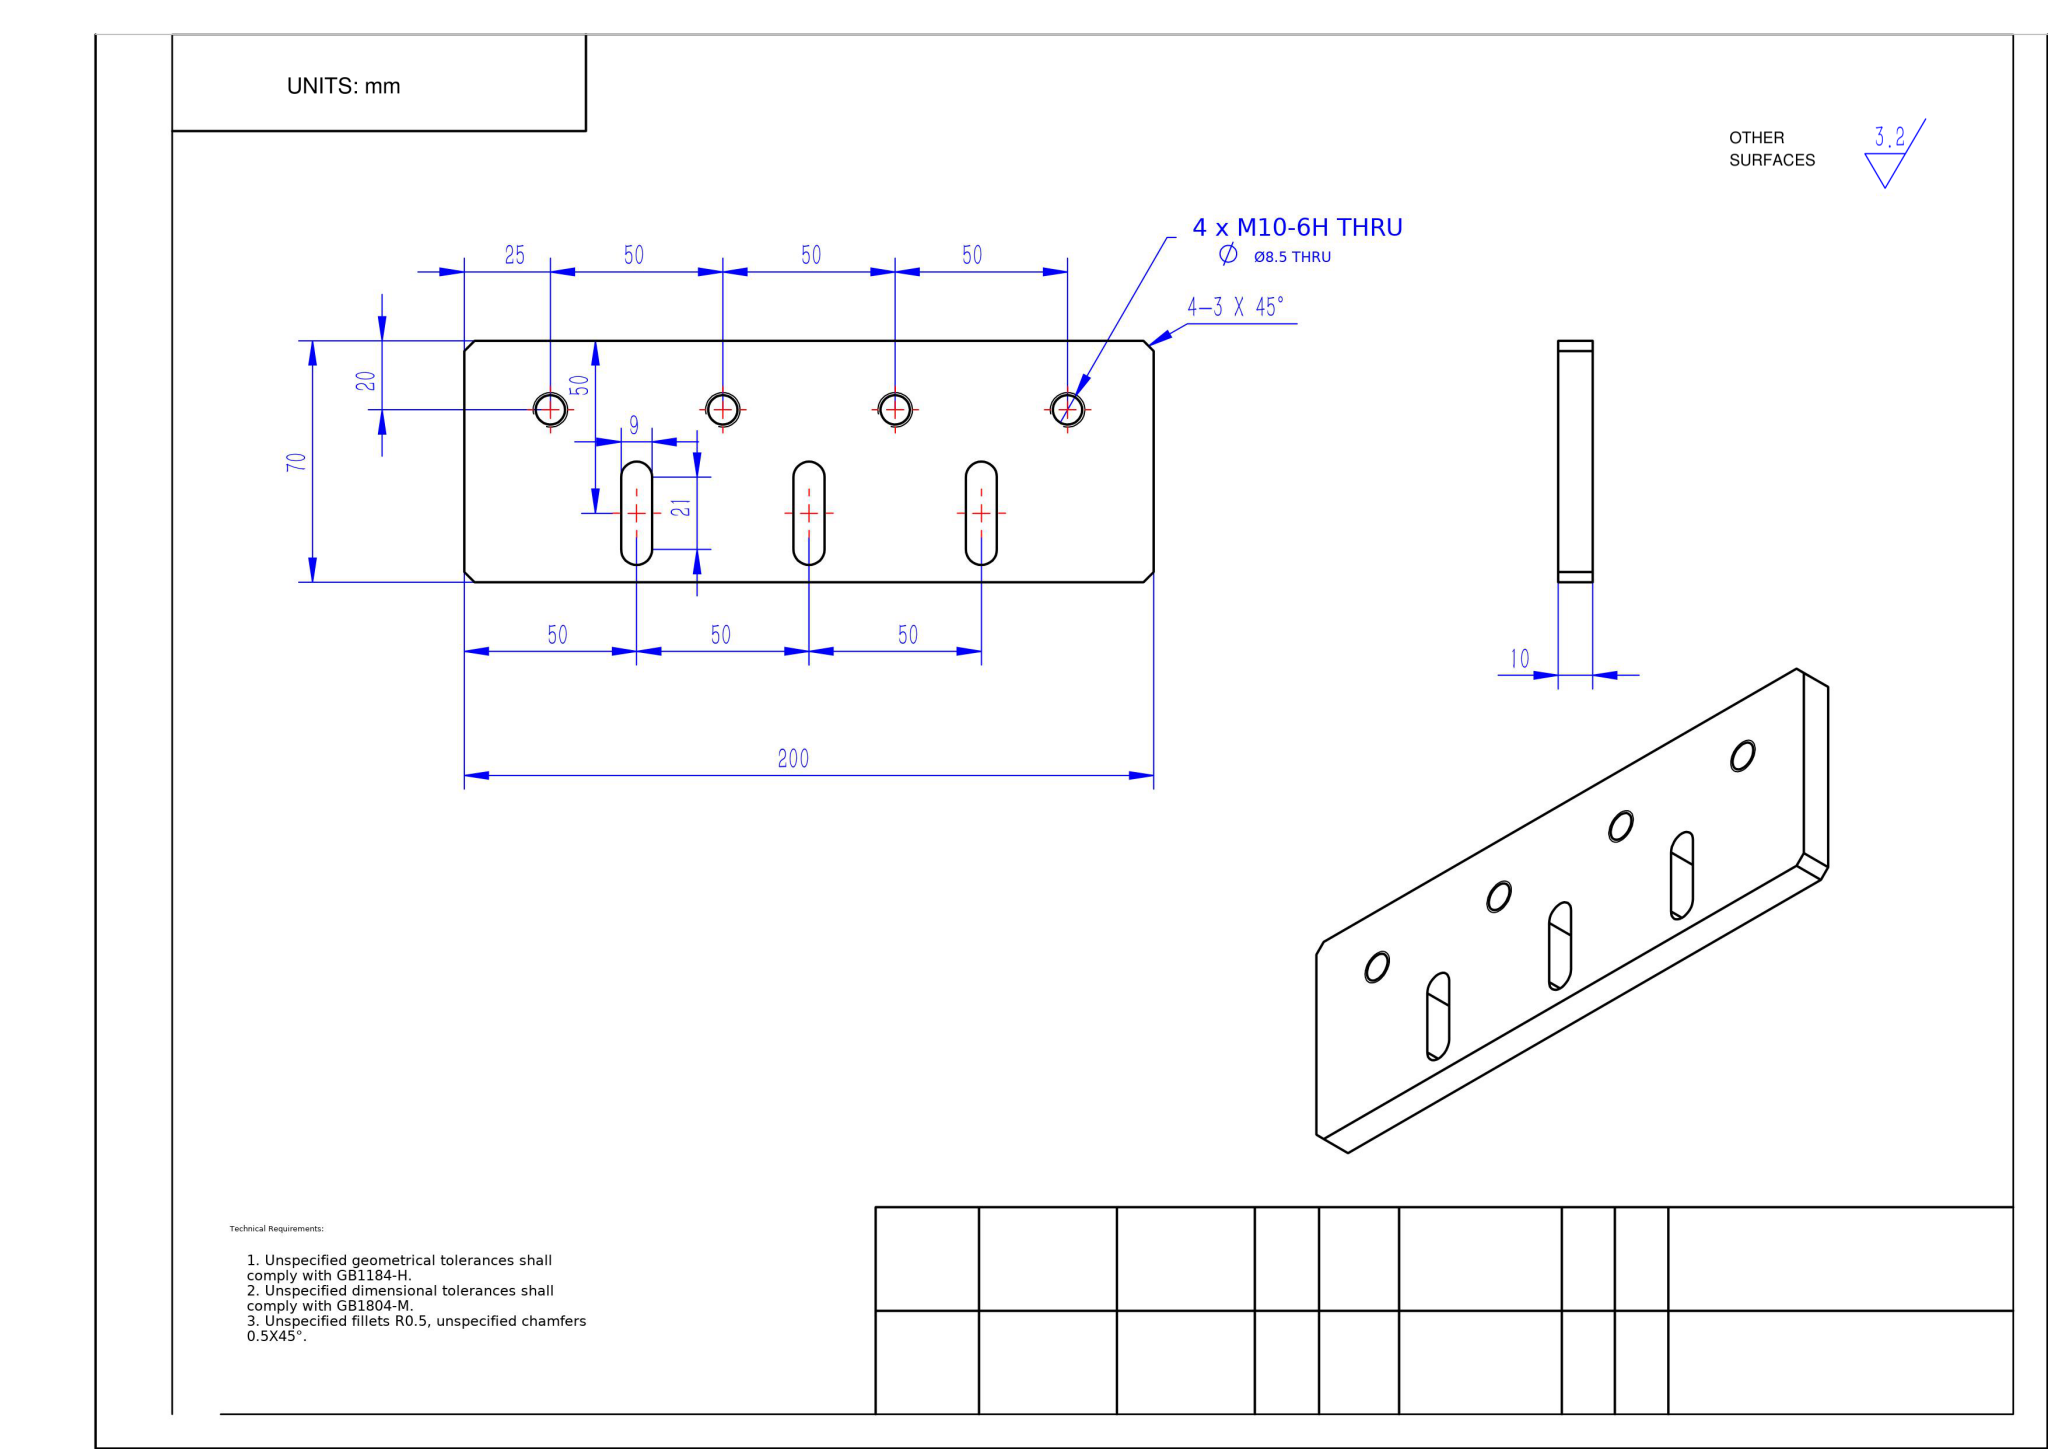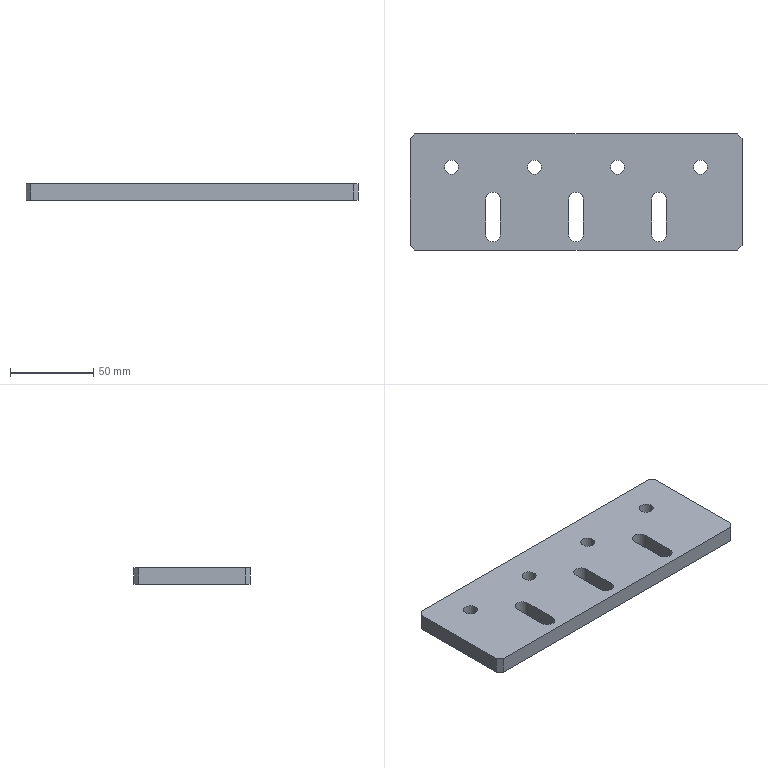Part | NX | mm | 1 solid | 30 faces | box 200 x 70 x 10 mm | volume 129972 mm3 | plane 16 | cylinder 14 | commonest cylinder face diameters 8.5 x8 9 x6